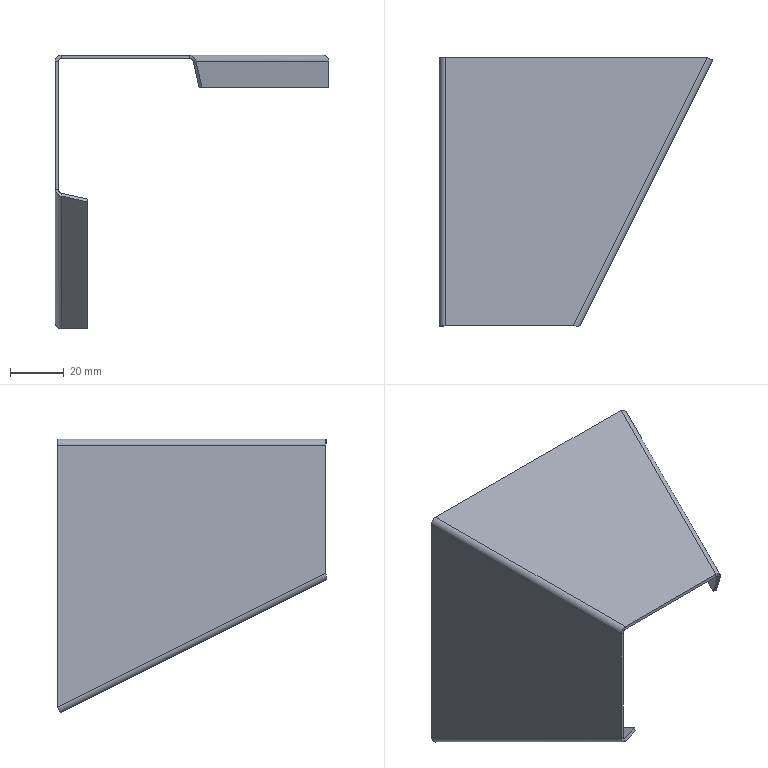Component | SolidWorks | BaseFoot-H100-1 | 1 solid | 30 faces | box 101.97 x 100.16 x 101.97 mm | volume 20988 mm3 | plane 22 | cylinder 6 | spline 2 | commonest cylinder face diameters 2 x3 4.4 x3
STEP:
#1=COLOUR_RGB('',0.7922,0.8196,0.9333);
#2=FILL_AREA_STYLE_COLOUR('',#1);
#3=FILL_AREA_STYLE('',(#2));
#4=SURFACE_STYLE_FILL_AREA(#3);
#5=SURFACE_SIDE_STYLE('',(#4));
#6=SURFACE_STYLE_USAGE(.BOTH.,#5);
#7=PRESENTATION_STYLE_ASSIGNMENT((#6));
#8=CARTESIAN_POINT('',(-19.685,0.,6.102));
#9=VERTEX_POINT('',#8);
#10=CARTESIAN_POINT('',(-19.685,-0.,9.953));
#11=VERTEX_POINT('',#10);
#12=CARTESIAN_POINT('',(-19.685,-0.,6.102));
#13=DIRECTION('',(0.,0.,1.));
#14=VECTOR('',#13,39.37);
#15=LINE('',#12,#14);
#16=EDGE_CURVE('',#9,#11,#15,.T.);
#17=ORIENTED_EDGE('',*,*,#16,.F.);
#18=CARTESIAN_POINT('',(-19.685,-3.937,8.071));
#19=VERTEX_POINT('',#18);
#20=CARTESIAN_POINT('',(-19.685,-3.15,7.677));
#21=DIRECTION('',(-0.,0.8944,-0.4472));
#22=VECTOR('',#21,39.37);
#23=LINE('',#20,#22);
#24=EDGE_CURVE('',#19,#9,#23,.T.);
#25=ORIENTED_EDGE('',*,*,#24,.F.);
#26=CARTESIAN_POINT('',(-19.685,-3.937,9.953));
#27=VERTEX_POINT('',#26);
#28=CARTESIAN_POINT('',(-19.685,-3.937,6.102));
#29=DIRECTION('',(0.,0.,1.));
#30=VECTOR('',#29,39.37);
#31=LINE('',#28,#30);
#32=EDGE_CURVE('',#19,#27,#31,.T.);
#33=ORIENTED_EDGE('',*,*,#32,.T.);
#34=CARTESIAN_POINT('',(-19.685,-3.937,9.953));
#35=DIRECTION('',(0.,1.,0.));
#36=VECTOR('',#35,39.37);
#37=LINE('',#34,#36);
#38=EDGE_CURVE('',#27,#11,#37,.T.);
#39=ORIENTED_EDGE('',*,*,#38,.T.);
#40=EDGE_LOOP('',(#17,#25,#33,#39));
#41=FACE_OUTER_BOUND('',#40,.T.);
#42=CARTESIAN_POINT('',(-19.685,-3.937,6.102));
#43=DIRECTION('',(-1.,0.,0.));
#44=DIRECTION('',(0.,0.,1.));
#45=AXIS2_PLACEMENT_3D('',#42,#43,#44);
#46=PLANE('',#45);
#47=ADVANCED_FACE('',(#41),#46,.T.);
#48=CARTESIAN_POINT('',(-19.638,-3.937,8.071));
#49=VERTEX_POINT('',#48);
#50=CARTESIAN_POINT('',(-19.638,0.,6.102));
#51=VERTEX_POINT('',#50);
#52=CARTESIAN_POINT('',(-19.638,-3.15,7.677));
#53=DIRECTION('',(-0.,0.8944,-0.4472));
#54=VECTOR('',#53,39.37);
#55=LINE('',#52,#54);
#56=EDGE_CURVE('',#49,#51,#55,.T.);
#57=ORIENTED_EDGE('',*,*,#56,.T.);
#58=CARTESIAN_POINT('',(-19.638,-0.,9.953));
#59=VERTEX_POINT('',#58);
#60=CARTESIAN_POINT('',(-19.638,-0.,6.102));
#61=DIRECTION('',(0.,0.,1.));
#62=VECTOR('',#61,39.37);
#63=LINE('',#60,#62);
#64=EDGE_CURVE('',#51,#59,#63,.T.);
#65=ORIENTED_EDGE('',*,*,#64,.T.);
#66=CARTESIAN_POINT('',(-19.638,-3.937,9.953));
#67=VERTEX_POINT('',#66);
#68=CARTESIAN_POINT('',(-19.638,-3.937,9.953));
#69=DIRECTION('',(0.,1.,0.));
#70=VECTOR('',#69,39.37);
#71=LINE('',#68,#70);
#72=EDGE_CURVE('',#67,#59,#71,.T.);
#73=ORIENTED_EDGE('',*,*,#72,.F.);
#74=CARTESIAN_POINT('',(-19.638,-3.937,6.102));
#75=DIRECTION('',(0.,0.,1.));
#76=VECTOR('',#75,39.37);
#77=LINE('',#74,#76);
#78=EDGE_CURVE('',#49,#67,#77,.T.);
#79=ORIENTED_EDGE('',*,*,#78,.F.);
#80=EDGE_LOOP('',(#57,#65,#73,#79));
#81=FACE_OUTER_BOUND('',#80,.T.);
#82=CARTESIAN_POINT('',(-19.638,-3.937,6.102));
#83=DIRECTION('',(-1.,0.,0.));
#84=DIRECTION('',(0.,0.,1.));
#85=AXIS2_PLACEMENT_3D('',#82,#83,#84);
#86=PLANE('',#85);
#87=ADVANCED_FACE('',(#81),#86,.F.);
#88=CARTESIAN_POINT('',(-19.638,-3.937,8.071));
#89=CARTESIAN_POINT('',(-19.685,-3.937,8.071));
#90=B_SPLINE_CURVE_WITH_KNOTS('',1,(#88,#89),.UNSPECIFIED.,.F.,.F.,(2,2),(0.,1.),.UNSPECIFIED.);
#91=EDGE_CURVE('',#49,#19,#90,.T.);
#92=ORIENTED_EDGE('',*,*,#91,.F.);
#93=ORIENTED_EDGE('',*,*,#78,.T.);
#94=CARTESIAN_POINT('',(-19.638,-3.937,9.953));
#95=DIRECTION('',(-1.,0.,0.));
#96=VECTOR('',#95,39.37);
#97=LINE('',#94,#96);
#98=EDGE_CURVE('',#67,#27,#97,.T.);
#99=ORIENTED_EDGE('',*,*,#98,.T.);
#100=ORIENTED_EDGE('',*,*,#32,.F.);
#101=EDGE_LOOP('',(#92,#93,#99,#100));
#102=FACE_OUTER_BOUND('',#101,.T.);
#103=CARTESIAN_POINT('',(-19.598,-3.937,9.953));
#104=DIRECTION('',(0.,1.,0.));
#105=DIRECTION('',(1.,0.,0.));
#106=AXIS2_PLACEMENT_3D('',#103,#104,#105);
#107=PLANE('',#106);
#108=ADVANCED_FACE('',(#102),#107,.F.);
#109=ORIENTED_EDGE('',*,*,#16,.T.);
#110=CARTESIAN_POINT('',(-19.685,-0.,9.953));
#111=DIRECTION('',(1.,0.,-0.));
#112=VECTOR('',#111,39.37);
#113=LINE('',#110,#112);
#114=EDGE_CURVE('',#11,#59,#113,.T.);
#115=ORIENTED_EDGE('',*,*,#114,.T.);
#116=ORIENTED_EDGE('',*,*,#64,.F.);
#117=CARTESIAN_POINT('',(-19.685,-0.,6.102));
#118=DIRECTION('',(1.,0.,0.));
#119=VECTOR('',#118,39.37);
#120=LINE('',#117,#119);
#121=EDGE_CURVE('',#9,#51,#120,.T.);
#122=ORIENTED_EDGE('',*,*,#121,.F.);
#123=EDGE_LOOP('',(#109,#115,#116,#122));
#124=FACE_OUTER_BOUND('',#123,.T.);
#125=CARTESIAN_POINT('',(-19.598,-0.,9.992));
#126=DIRECTION('',(0.,1.,0.));
#127=DIRECTION('',(0.,0.,1.));
#128=AXIS2_PLACEMENT_3D('',#125,#126,#127);
#129=PLANE('',#128);
#130=ADVANCED_FACE('',(#124),#129,.T.);
#131=CARTESIAN_POINT('',(-17.717,-3.937,9.992));
#132=VERTEX_POINT('',#131);
#133=CARTESIAN_POINT('',(-15.748,-0.,9.992));
#134=VERTEX_POINT('',#133);
#135=CARTESIAN_POINT('',(-18.11,-4.724,9.992));
#136=DIRECTION('',(0.4472,0.8944,0.));
#137=VECTOR('',#136,39.37);
#138=LINE('',#135,#137);
#139=EDGE_CURVE('',#132,#134,#138,.T.);
#140=ORIENTED_EDGE('',*,*,#139,.F.);
#141=CARTESIAN_POINT('',(-19.598,-3.937,9.992));
#142=VERTEX_POINT('',#141);
#143=CARTESIAN_POINT('',(-19.685,-3.937,9.992));
#144=DIRECTION('',(1.,0.,0.));
#145=VECTOR('',#144,39.37);
#146=LINE('',#143,#145);
#147=EDGE_CURVE('',#142,#132,#146,.T.);
#148=ORIENTED_EDGE('',*,*,#147,.F.);
#149=CARTESIAN_POINT('',(-19.598,-0.,9.992));
#150=VERTEX_POINT('',#149);
#151=CARTESIAN_POINT('',(-19.598,-3.937,9.992));
#152=DIRECTION('',(0.,1.,0.));
#153=VECTOR('',#152,39.37);
#154=LINE('',#151,#153);
#155=EDGE_CURVE('',#142,#150,#154,.T.);
#156=ORIENTED_EDGE('',*,*,#155,.T.);
#157=CARTESIAN_POINT('',(-19.685,-0.,9.992));
#158=DIRECTION('',(1.,0.,0.));
#159=VECTOR('',#158,39.37);
#160=LINE('',#157,#159);
#161=EDGE_CURVE('',#150,#134,#160,.T.);
#162=ORIENTED_EDGE('',*,*,#161,.T.);
#163=EDGE_LOOP('',(#140,#148,#156,#162));
#164=FACE_OUTER_BOUND('',#163,.T.);
#165=CARTESIAN_POINT('',(-19.685,-3.937,9.992));
#166=DIRECTION('',(0.,0.,1.));
#167=DIRECTION('',(1.,0.,0.));
#168=AXIS2_PLACEMENT_3D('',#165,#166,#167);
#169=PLANE('',#168);
#170=ADVANCED_FACE('',(#164),#169,.F.);
#171=CARTESIAN_POINT('',(-19.598,-0.,10.039));
#172=VERTEX_POINT('',#171);
#173=CARTESIAN_POINT('',(-15.748,-0.,10.039));
#174=VERTEX_POINT('',#173);
#175=CARTESIAN_POINT('',(-19.685,-0.,10.039));
#176=DIRECTION('',(1.,0.,0.));
#177=VECTOR('',#176,39.37);
#178=LINE('',#175,#177);
#179=EDGE_CURVE('',#172,#174,#178,.T.);
#180=ORIENTED_EDGE('',*,*,#179,.T.);
#181=CARTESIAN_POINT('',(-15.748,-0.,9.992));
#182=DIRECTION('',(0.,0.,1.));
#183=VECTOR('',#182,39.37);
#184=LINE('',#181,#183);
#185=EDGE_CURVE('',#134,#174,#184,.T.);
#186=ORIENTED_EDGE('',*,*,#185,.F.);
#187=ORIENTED_EDGE('',*,*,#161,.F.);
#188=CARTESIAN_POINT('',(-19.598,-0.,9.992));
#189=DIRECTION('',(0.,0.,1.));
#190=VECTOR('',#189,39.37);
#191=LINE('',#188,#190);
#192=EDGE_CURVE('',#150,#172,#191,.T.);
#193=ORIENTED_EDGE('',*,*,#192,.T.);
#194=EDGE_LOOP('',(#180,#186,#187,#193));
#195=FACE_OUTER_BOUND('',#194,.T.);
#196=CARTESIAN_POINT('',(-19.598,-0.,9.953));
#197=DIRECTION('',(0.,1.,0.));
#198=DIRECTION('',(1.,0.,0.));
#199=AXIS2_PLACEMENT_3D('',#196,#197,#198);
#200=PLANE('',#199);
#201=ADVANCED_FACE('',(#195),#200,.T.);
#202=CARTESIAN_POINT('',(-19.598,-3.937,10.039));
#203=VERTEX_POINT('',#202);
#204=CARTESIAN_POINT('',(-17.717,-3.937,10.039));
#205=VERTEX_POINT('',#204);
#206=CARTESIAN_POINT('',(-19.685,-3.937,10.039));
#207=DIRECTION('',(1.,0.,0.));
#208=VECTOR('',#207,39.37);
#209=LINE('',#206,#208);
#210=EDGE_CURVE('',#203,#205,#209,.T.);
#211=ORIENTED_EDGE('',*,*,#210,.T.);
#212=CARTESIAN_POINT('',(-18.11,-4.724,10.039));
#213=DIRECTION('',(0.4472,0.8944,0.));
#214=VECTOR('',#213,39.37);
#215=LINE('',#212,#214);
#216=EDGE_CURVE('',#205,#174,#215,.T.);
#217=ORIENTED_EDGE('',*,*,#216,.T.);
#218=ORIENTED_EDGE('',*,*,#179,.F.);
#219=CARTESIAN_POINT('',(-19.598,-3.937,10.039));
#220=DIRECTION('',(0.,1.,0.));
#221=VECTOR('',#220,39.37);
#222=LINE('',#219,#221);
#223=EDGE_CURVE('',#203,#172,#222,.T.);
#224=ORIENTED_EDGE('',*,*,#223,.F.);
#225=EDGE_LOOP('',(#211,#217,#218,#224));
#226=FACE_OUTER_BOUND('',#225,.T.);
#227=CARTESIAN_POINT('',(-19.685,-3.937,10.039));
#228=DIRECTION('',(0.,0.,1.));
#229=DIRECTION('',(1.,0.,0.));
#230=AXIS2_PLACEMENT_3D('',#227,#228,#229);
#231=PLANE('',#230);
#232=ADVANCED_FACE('',(#226),#231,.T.);
#233=ORIENTED_EDGE('',*,*,#147,.T.);
#234=CARTESIAN_POINT('',(-17.717,-3.937,10.039));
#235=CARTESIAN_POINT('',(-17.717,-3.937,9.992));
#236=B_SPLINE_CURVE_WITH_KNOTS('',1,(#234,#235),.UNSPECIFIED.,.F.,.F.,(2,2),(0.,1.),.UNSPECIFIED.);
#237=EDGE_CURVE('',#205,#132,#236,.T.);
#238=ORIENTED_EDGE('',*,*,#237,.F.);
#239=ORIENTED_EDGE('',*,*,#210,.F.);
#240=CARTESIAN_POINT('',(-19.598,-3.937,10.039));
#241=DIRECTION('',(0.,0.,-1.));
#242=VECTOR('',#241,39.37);
#243=LINE('',#240,#242);
#244=EDGE_CURVE('',#203,#142,#243,.T.);
#245=ORIENTED_EDGE('',*,*,#244,.T.);
#246=EDGE_LOOP('',(#233,#238,#239,#245));
#247=FACE_OUTER_BOUND('',#246,.T.);
#248=CARTESIAN_POINT('',(-19.638,-3.937,9.953));
#249=DIRECTION('',(0.,-1.,0.));
#250=DIRECTION('',(0.,0.,-1.));
#251=AXIS2_PLACEMENT_3D('',#248,#249,#250);
#252=PLANE('',#251);
#253=ADVANCED_FACE('',(#247),#252,.T.);
#254=ORIENTED_EDGE('',*,*,#244,.F.);
#255=CARTESIAN_POINT('',(-19.598,-3.937,9.953));
#256=DIRECTION('',(0.,-1.,0.));
#257=DIRECTION('',(0.,0.,1.));
#258=AXIS2_PLACEMENT_3D('',#255,#256,#257);
#259=CIRCLE('',#258,0.08661);
#260=EDGE_CURVE('',#203,#27,#259,.T.);
#261=ORIENTED_EDGE('',*,*,#260,.T.);
#262=ORIENTED_EDGE('',*,*,#98,.F.);
#263=CARTESIAN_POINT('',(-19.598,-3.937,9.953));
#264=DIRECTION('',(0.,-1.,0.));
#265=DIRECTION('',(0.,0.,-1.));
#266=AXIS2_PLACEMENT_3D('',#263,#264,#265);
#267=CIRCLE('',#266,0.03937);
#268=EDGE_CURVE('',#142,#67,#267,.T.);
#269=ORIENTED_EDGE('',*,*,#268,.F.);
#270=EDGE_LOOP('',(#254,#261,#262,#269));
#271=FACE_OUTER_BOUND('',#270,.T.);
#272=CARTESIAN_POINT('',(-19.598,-3.937,9.953));
#273=DIRECTION('',(0.,1.,0.));
#274=DIRECTION('',(0.,0.,1.));
#275=AXIS2_PLACEMENT_3D('',#272,#273,#274);
#276=PLANE('',#275);
#277=ADVANCED_FACE('',(#271),#276,.F.);
#278=ORIENTED_EDGE('',*,*,#114,.F.);
#279=CARTESIAN_POINT('',(-19.598,-0.,9.953));
#280=DIRECTION('',(0.,1.,0.));
#281=DIRECTION('',(0.,0.,1.));
#282=AXIS2_PLACEMENT_3D('',#279,#280,#281);
#283=CIRCLE('',#282,0.08661);
#284=EDGE_CURVE('',#11,#172,#283,.T.);
#285=ORIENTED_EDGE('',*,*,#284,.T.);
#286=ORIENTED_EDGE('',*,*,#192,.F.);
#287=CARTESIAN_POINT('',(-19.598,-0.,9.953));
#288=DIRECTION('',(0.,1.,0.));
#289=DIRECTION('',(0.,0.,1.));
#290=AXIS2_PLACEMENT_3D('',#287,#288,#289);
#291=CIRCLE('',#290,0.03937);
#292=EDGE_CURVE('',#59,#150,#291,.T.);
#293=ORIENTED_EDGE('',*,*,#292,.F.);
#294=EDGE_LOOP('',(#278,#285,#286,#293));
#295=FACE_OUTER_BOUND('',#294,.T.);
#296=CARTESIAN_POINT('',(-19.598,-0.,9.953));
#297=DIRECTION('',(0.,-1.,0.));
#298=DIRECTION('',(0.,0.,-1.));
#299=AXIS2_PLACEMENT_3D('',#296,#297,#298);
#300=PLANE('',#299);
#301=ADVANCED_FACE('',(#295),#300,.F.);
#302=ORIENTED_EDGE('',*,*,#292,.T.);
#303=ORIENTED_EDGE('',*,*,#155,.F.);
#304=ORIENTED_EDGE('',*,*,#268,.T.);
#305=ORIENTED_EDGE('',*,*,#72,.T.);
#306=EDGE_LOOP('',(#302,#303,#304,#305));
#307=FACE_OUTER_BOUND('',#306,.T.);
#308=CARTESIAN_POINT('',(-19.598,-5.907,9.953));
#309=DIRECTION('',(0.,1.,0.));
#310=DIRECTION('',(0.,0.,1.));
#311=AXIS2_PLACEMENT_3D('',#308,#309,#310);
#312=CYLINDRICAL_SURFACE('',#311,0.03937);
#313=ADVANCED_FACE('',(#307),#312,.F.);
#314=ORIENTED_EDGE('',*,*,#284,.F.);
#315=ORIENTED_EDGE('',*,*,#38,.F.);
#316=ORIENTED_EDGE('',*,*,#260,.F.);
#317=ORIENTED_EDGE('',*,*,#223,.T.);
#318=EDGE_LOOP('',(#314,#315,#316,#317));
#319=FACE_OUTER_BOUND('',#318,.T.);
#320=CARTESIAN_POINT('',(-19.598,-5.907,9.953));
#321=DIRECTION('',(0.,1.,0.));
#322=DIRECTION('',(0.,0.,1.));
#323=AXIS2_PLACEMENT_3D('',#320,#321,#322);
#324=CYLINDRICAL_SURFACE('',#323,0.08661);
#325=ADVANCED_FACE('',(#319),#324,.T.);
#326=CARTESIAN_POINT('',(-17.618,-3.933,9.953));
#327=VERTEX_POINT('',#326);
#328=CARTESIAN_POINT('',(-17.66,-3.912,9.953));
#329=VERTEX_POINT('',#328);
#330=CARTESIAN_POINT('',(-17.618,-3.933,9.953));
#331=CARTESIAN_POINT('',(-17.632,-3.926,9.953));
#332=CARTESIAN_POINT('',(-17.646,-3.919,9.953));
#333=CARTESIAN_POINT('',(-17.66,-3.912,9.953));
#334=B_SPLINE_CURVE_WITH_KNOTS('',3,(#330,#331,#332,#333),.UNSPECIFIED.,.F.,.F.,(4,4),(0.,1.),.UNSPECIFIED.);
#335=EDGE_CURVE('',#327,#329,#334,.T.);
#336=ORIENTED_EDGE('',*,*,#335,.F.);
#337=CARTESIAN_POINT('',(-17.618,-3.933,9.953));
#338=CARTESIAN_POINT('',(-17.62,-3.937,9.964));
#339=CARTESIAN_POINT('',(-17.623,-3.94,9.975));
#340=CARTESIAN_POINT('',(-17.635,-3.943,9.996));
#341=CARTESIAN_POINT('',(-17.642,-3.943,10.006));
#342=CARTESIAN_POINT('',(-17.66,-3.943,10.022));
#343=CARTESIAN_POINT('',(-17.67,-3.942,10.028));
#344=CARTESIAN_POINT('',(-17.693,-3.94,10.037));
#345=CARTESIAN_POINT('',(-17.705,-3.939,10.039));
#346=CARTESIAN_POINT('',(-17.717,-3.937,10.039));
#347=B_SPLINE_CURVE_WITH_KNOTS('',3,(#337,#338,#339,#340,#341,#342,#343,#344,#345,#346),.UNSPECIFIED.,.F.,.F.,(4,2,2,2,4),(0.,0.25,0.5,0.75,1.),.UNSPECIFIED.);
#348=EDGE_CURVE('',#327,#205,#347,.T.);
#349=ORIENTED_EDGE('',*,*,#348,.T.);
#350=ORIENTED_EDGE('',*,*,#237,.T.);
#351=CARTESIAN_POINT('',(-17.66,-3.912,9.953));
#352=CARTESIAN_POINT('',(-17.664,-3.919,9.963));
#353=CARTESIAN_POINT('',(-17.671,-3.925,9.973));
#354=CARTESIAN_POINT('',(-17.691,-3.932,9.988));
#355=CARTESIAN_POINT('',(-17.704,-3.935,9.992));
#356=CARTESIAN_POINT('',(-17.717,-3.937,9.992));
#357=B_SPLINE_CURVE_WITH_KNOTS('',3,(#351,#352,#353,#354,#355,#356),.UNSPECIFIED.,.F.,.F.,(4,2,4),(0.,0.5,1.),.UNSPECIFIED.);
#358=EDGE_CURVE('',#329,#132,#357,.T.);
#359=ORIENTED_EDGE('',*,*,#358,.F.);
#360=EDGE_LOOP('',(#336,#349,#350,#359));
#361=FACE_OUTER_BOUND('',#360,.T.);
#362=CARTESIAN_POINT('',(-17.618,-3.933,9.953));
#363=CARTESIAN_POINT('',(-17.62,-3.937,9.964));
#364=CARTESIAN_POINT('',(-17.623,-3.94,9.975));
#365=CARTESIAN_POINT('',(-17.635,-3.943,9.996));
#366=CARTESIAN_POINT('',(-17.642,-3.943,10.006));
#367=CARTESIAN_POINT('',(-17.66,-3.943,10.022));
#368=CARTESIAN_POINT('',(-17.67,-3.942,10.028));
#369=CARTESIAN_POINT('',(-17.693,-3.94,10.037));
#370=CARTESIAN_POINT('',(-17.705,-3.939,10.039));
#371=CARTESIAN_POINT('',(-17.717,-3.937,10.039));
#372=CARTESIAN_POINT('',(-17.66,-3.912,9.953));
#373=CARTESIAN_POINT('',(-17.662,-3.916,9.958));
#374=CARTESIAN_POINT('',(-17.665,-3.919,9.963));
#375=CARTESIAN_POINT('',(-17.672,-3.924,9.973));
#376=CARTESIAN_POINT('',(-17.676,-3.926,9.977));
#377=CARTESIAN_POINT('',(-17.686,-3.93,9.984));
#378=CARTESIAN_POINT('',(-17.692,-3.932,9.987));
#379=CARTESIAN_POINT('',(-17.704,-3.935,9.991));
#380=CARTESIAN_POINT('',(-17.71,-3.936,9.992));
#381=CARTESIAN_POINT('',(-17.717,-3.937,9.992));
#382=B_SPLINE_SURFACE_WITH_KNOTS('',1,3,((#362,#363,#364,#365,#366,#367,#368,#369,#370,#371),(#372,#373,#374,#375,#376,#377,#378,#379,#380,#381)),.UNSPECIFIED.,.F.,.F.,.F.,(2,2),(4,2,2,2,4),(0.,1.),(0.,0.25,0.5,0.75,1.),.UNSPECIFIED.);
#383=ADVANCED_FACE('',(#361),#382,.F.);
#384=CARTESIAN_POINT('',(-15.671,-0.03874,9.953));
#385=VERTEX_POINT('',#384);
#386=CARTESIAN_POINT('',(-15.748,0.,9.953));
#387=DIRECTION('',(0.4472,0.8944,0.));
#388=DIRECTION('',(0.8944,-0.4472,0.));
#389=AXIS2_PLACEMENT_3D('',#386,#387,#388);
#390=CIRCLE('',#389,0.08661);
#391=EDGE_CURVE('',#174,#385,#390,.T.);
#392=ORIENTED_EDGE('',*,*,#391,.T.);
#393=CARTESIAN_POINT('',(-15.713,-0.01761,9.953));
#394=VERTEX_POINT('',#393);
#395=CARTESIAN_POINT('',(-15.671,-0.03874,9.953));
#396=DIRECTION('',(0.8944,-0.4472,0.));
#397=VECTOR('',#396,39.37);
#398=LINE('',#395,#397);
#399=EDGE_CURVE('',#394,#385,#398,.T.);
#400=ORIENTED_EDGE('',*,*,#399,.F.);
#401=CARTESIAN_POINT('',(-15.748,0.,9.953));
#402=DIRECTION('',(0.4472,0.8944,0.));
#403=DIRECTION('',(-0.8944,0.4472,0.));
#404=AXIS2_PLACEMENT_3D('',#401,#402,#403);
#405=CIRCLE('',#404,0.03937);
#406=EDGE_CURVE('',#134,#394,#405,.T.);
#407=ORIENTED_EDGE('',*,*,#406,.F.);
#408=ORIENTED_EDGE('',*,*,#185,.T.);
#409=EDGE_LOOP('',(#392,#400,#407,#408));
#410=FACE_OUTER_BOUND('',#409,.T.);
#411=CARTESIAN_POINT('',(-15.748,0.,9.953));
#412=DIRECTION('',(-0.4472,-0.8944,-0.));
#413=DIRECTION('',(0.8944,-0.4472,0.));
#414=AXIS2_PLACEMENT_3D('',#411,#412,#413);
#415=PLANE('',#414);
#416=ADVANCED_FACE('',(#410),#415,.F.);
#417=ORIENTED_EDGE('',*,*,#139,.T.);
#418=ORIENTED_EDGE('',*,*,#406,.T.);
#419=CARTESIAN_POINT('',(-15.713,-0.01761,9.953));
#420=DIRECTION('',(-0.4472,-0.8944,0.));
#421=VECTOR('',#420,39.37);
#422=LINE('',#419,#421);
#423=EDGE_CURVE('',#394,#329,#422,.T.);
#424=ORIENTED_EDGE('',*,*,#423,.T.);
#425=ORIENTED_EDGE('',*,*,#358,.T.);
#426=EDGE_LOOP('',(#417,#418,#424,#425));
#427=FACE_OUTER_BOUND('',#426,.T.);
#428=CARTESIAN_POINT('',(-14.746,2.003,9.953));
#429=DIRECTION('',(-0.4472,-0.8944,0.));
#430=DIRECTION('',(0.8944,-0.4472,0.));
#431=AXIS2_PLACEMENT_3D('',#428,#429,#430);
#432=CYLINDRICAL_SURFACE('',#431,0.03937);
#433=ADVANCED_FACE('',(#427),#432,.F.);
#434=ORIENTED_EDGE('',*,*,#216,.F.);
#435=ORIENTED_EDGE('',*,*,#348,.F.);
#436=CARTESIAN_POINT('',(-16.458,-1.614,9.953));
#437=DIRECTION('',(-0.4472,-0.8944,0.));
#438=VECTOR('',#437,39.37);
#439=LINE('',#436,#438);
#440=EDGE_CURVE('',#385,#327,#439,.T.);
#441=ORIENTED_EDGE('',*,*,#440,.F.);
#442=ORIENTED_EDGE('',*,*,#391,.F.);
#443=EDGE_LOOP('',(#434,#435,#441,#442));
#444=FACE_OUTER_BOUND('',#443,.T.);
#445=CARTESIAN_POINT('',(-14.746,2.003,9.953));
#446=DIRECTION('',(-0.4472,-0.8944,0.));
#447=DIRECTION('',(0.8944,-0.4472,0.));
#448=AXIS2_PLACEMENT_3D('',#445,#446,#447);
#449=CYLINDRICAL_SURFACE('',#448,0.08661);
#450=ADVANCED_FACE('',(#444),#449,.T.);
#451=CARTESIAN_POINT('',(-15.671,-0.03874,9.567));
#452=VERTEX_POINT('',#451);
#453=CARTESIAN_POINT('',(-17.532,-3.761,9.567));
#454=VERTEX_POINT('',#453);
#455=CARTESIAN_POINT('',(-17.639,-3.976,9.567));
#456=DIRECTION('',(-0.4472,-0.8944,0.));
#457=VECTOR('',#456,39.37);
#458=LINE('',#455,#457);
#459=EDGE_CURVE('',#452,#454,#458,.T.);
#460=ORIENTED_EDGE('',*,*,#459,.T.);
#461=CARTESIAN_POINT('',(-17.574,-3.74,9.567));
#462=VERTEX_POINT('',#461);
#463=CARTESIAN_POINT('',(-17.532,-3.761,9.567));
#464=DIRECTION('',(-0.8944,0.4472,-0.));
#465=VECTOR('',#464,39.37);
#466=LINE('',#463,#465);
#467=EDGE_CURVE('',#454,#462,#466,.T.);
#468=ORIENTED_EDGE('',*,*,#467,.T.);
#469=CARTESIAN_POINT('',(-15.713,-0.01761,9.567));
#470=VERTEX_POINT('',#469);
#471=CARTESIAN_POINT('',(-16.5,-1.592,9.567));
#472=DIRECTION('',(-0.4472,-0.8944,0.));
#473=VECTOR('',#472,39.37);
#474=LINE('',#471,#473);
#475=EDGE_CURVE('',#470,#462,#474,.T.);
#476=ORIENTED_EDGE('',*,*,#475,.F.);
#477=CARTESIAN_POINT('',(-15.671,-0.03874,9.567));
#478=DIRECTION('',(-0.8944,0.4472,-0.));
#479=VECTOR('',#478,39.37);
#480=LINE('',#477,#479);
#481=EDGE_CURVE('',#452,#470,#480,.T.);
#482=ORIENTED_EDGE('',*,*,#481,.F.);
#483=EDGE_LOOP('',(#460,#468,#476,#482));
#484=FACE_OUTER_BOUND('',#483,.T.);
#485=CARTESIAN_POINT('',(-17.639,-3.976,9.567));
#486=DIRECTION('',(0.,-0.,-1.));
#487=DIRECTION('',(-1.,-0.,-0.));
#488=AXIS2_PLACEMENT_3D('',#485,#486,#487);
#489=PLANE('',#488);
#490=ADVANCED_FACE('',(#484),#489,.T.);
#491=CARTESIAN_POINT('',(-17.444,-3.479,8.985));
#492=DIRECTION('',(-0.2,-0.4,0.8944));
#493=VECTOR('',#492,39.37);
#494=LINE('',#491,#493);
#495=EDGE_CURVE('',#462,#329,#494,.T.);
#496=ORIENTED_EDGE('',*,*,#495,.T.);
#497=ORIENTED_EDGE('',*,*,#423,.F.);
#498=CARTESIAN_POINT('',(-15.713,-0.01761,10.039));
#499=DIRECTION('',(0.,0.,-1.));
#500=VECTOR('',#499,39.37);
#501=LINE('',#498,#500);
#502=EDGE_CURVE('',#394,#470,#501,.T.);
#503=ORIENTED_EDGE('',*,*,#502,.T.);
#504=ORIENTED_EDGE('',*,*,#475,.T.);
#505=EDGE_LOOP('',(#496,#497,#503,#504));
#506=FACE_OUTER_BOUND('',#505,.T.);
#507=CARTESIAN_POINT('',(-16.5,-1.592,10.039));
#508=DIRECTION('',(0.8944,-0.4472,0.));
#509=DIRECTION('',(0.4472,0.8944,-0.));
#510=AXIS2_PLACEMENT_3D('',#507,#508,#509);
#511=PLANE('',#510);
#512=ADVANCED_FACE('',(#506),#511,.F.);
#513=ORIENTED_EDGE('',*,*,#502,.F.);
#514=ORIENTED_EDGE('',*,*,#399,.T.);
#515=CARTESIAN_POINT('',(-15.671,-0.03874,9.567));
#516=DIRECTION('',(0.,0.,-1.));
#517=VECTOR('',#516,39.37);
#518=LINE('',#515,#517);
#519=EDGE_CURVE('',#385,#452,#518,.T.);
#520=ORIENTED_EDGE('',*,*,#519,.T.);
#521=ORIENTED_EDGE('',*,*,#481,.T.);
#522=EDGE_LOOP('',(#513,#514,#520,#521));
#523=FACE_OUTER_BOUND('',#522,.T.);
#524=CARTESIAN_POINT('',(-15.671,-0.03874,9.567));
#525=DIRECTION('',(0.4472,0.8944,0.));
#526=DIRECTION('',(-0.8944,0.4472,-0.));
#527=AXIS2_PLACEMENT_3D('',#524,#525,#526);
#528=PLANE('',#527);
#529=ADVANCED_FACE('',(#523),#528,.T.);
#530=ORIENTED_EDGE('',*,*,#440,.T.);
#531=CARTESIAN_POINT('',(-17.401,-3.5,8.985));
#532=DIRECTION('',(-0.2,-0.4,0.8944));
#533=VECTOR('',#532,39.37);
#534=LINE('',#531,#533);
#535=EDGE_CURVE('',#454,#327,#534,.T.);
#536=ORIENTED_EDGE('',*,*,#535,.F.);
#537=ORIENTED_EDGE('',*,*,#459,.F.);
#538=ORIENTED_EDGE('',*,*,#519,.F.);
#539=EDGE_LOOP('',(#530,#536,#537,#538));
#540=FACE_OUTER_BOUND('',#539,.T.);
#541=CARTESIAN_POINT('',(-16.458,-1.614,10.039));
#542=DIRECTION('',(0.8944,-0.4472,0.));
#543=DIRECTION('',(0.4472,0.8944,-0.));
#544=AXIS2_PLACEMENT_3D('',#541,#542,#543);
#545=PLANE('',#544);
#546=ADVANCED_FACE('',(#540),#545,.T.);
#547=ORIENTED_EDGE('',*,*,#535,.T.);
#548=ORIENTED_EDGE('',*,*,#335,.T.);
#549=ORIENTED_EDGE('',*,*,#495,.F.);
#550=ORIENTED_EDGE('',*,*,#467,.F.);
#551=EDGE_LOOP('',(#547,#548,#549,#550));
#552=FACE_OUTER_BOUND('',#551,.T.);
#553=CARTESIAN_POINT('',(-17.401,-3.5,8.985));
#554=DIRECTION('',(0.4,0.8,0.4472));
#555=DIRECTION('',(-0.2,-0.4,0.8944));
#556=AXIS2_PLACEMENT_3D('',#553,#554,#555);
#557=PLANE('',#556);
#558=ADVANCED_FACE('',(#552),#557,.F.);
#559=ORIENTED_EDGE('',*,*,#91,.T.);
#560=CARTESIAN_POINT('',(-19.598,-3.933,7.972));
#561=VERTEX_POINT('',#560);
#562=CARTESIAN_POINT('',(-19.685,-3.937,8.071));
#563=CARTESIAN_POINT('',(-19.685,-3.939,8.059));
#564=CARTESIAN_POINT('',(-19.683,-3.94,8.047));
#565=CARTESIAN_POINT('',(-19.674,-3.942,8.025));
#566=CARTESIAN_POINT('',(-19.668,-3.943,8.014));
#567=CARTESIAN_POINT('',(-19.652,-3.943,7.997));
#568=CARTESIAN_POINT('',(-19.642,-3.943,7.989));
#569=CARTESIAN_POINT('',(-19.621,-3.94,7.978));
#570=CARTESIAN_POINT('',(-19.61,-3.937,7.974));
#571=CARTESIAN_POINT('',(-19.598,-3.933,7.972));
#572=B_SPLINE_CURVE_WITH_KNOTS('',3,(#562,#563,#564,#565,#566,#567,#568,#569,#570,#571),.UNSPECIFIED.,.F.,.F.,(4,2,2,2,4),(0.,0.25,0.5,0.75,1.),.UNSPECIFIED.);
#573=EDGE_CURVE('',#19,#561,#572,.T.);
#574=ORIENTED_EDGE('',*,*,#573,.T.);
#575=CARTESIAN_POINT('',(-19.598,-3.912,8.015));
#576=VERTEX_POINT('',#575);
#577=CARTESIAN_POINT('',(-19.598,-3.912,8.015));
#578=CARTESIAN_POINT('',(-19.598,-3.919,8.));
#579=CARTESIAN_POINT('',(-19.598,-3.926,7.986));
#580=CARTESIAN_POINT('',(-19.598,-3.933,7.972));
#581=B_SPLINE_CURVE_WITH_KNOTS('',3,(#577,#578,#579,#580),.UNSPECIFIED.,.F.,.F.,(4,4),(0.,1.),.UNSPECIFIED.);
#582=EDGE_CURVE('',#576,#561,#581,.T.);
#583=ORIENTED_EDGE('',*,*,#582,.F.);
#584=CARTESIAN_POINT('',(-19.638,-3.937,8.071));
#585=CARTESIAN_POINT('',(-19.638,-3.935,8.058));
#586=CARTESIAN_POINT('',(-19.634,-3.932,8.045));
#587=CARTESIAN_POINT('',(-19.619,-3.925,8.025));
#588=CARTESIAN_POINT('',(-19.609,-3.919,8.018));
#589=CARTESIAN_POINT('',(-19.598,-3.912,8.015));
#590=B_SPLINE_CURVE_WITH_KNOTS('',3,(#584,#585,#586,#587,#588,#589),.UNSPECIFIED.,.F.,.F.,(4,2,4),(0.,0.5,1.),.UNSPECIFIED.);
#591=EDGE_CURVE('',#49,#576,#590,.T.);
#592=ORIENTED_EDGE('',*,*,#591,.F.);
#593=EDGE_LOOP('',(#559,#574,#583,#592));
#594=FACE_OUTER_BOUND('',#593,.T.);
#595=CARTESIAN_POINT('',(-19.685,-3.937,8.071));
#596=CARTESIAN_POINT('',(-19.685,-3.939,8.059));
#597=CARTESIAN_POINT('',(-19.683,-3.94,8.047));
#598=CARTESIAN_POINT('',(-19.674,-3.942,8.025));
#599=CARTESIAN_POINT('',(-19.668,-3.943,8.014));
#600=CARTESIAN_POINT('',(-19.652,-3.943,7.997));
#601=CARTESIAN_POINT('',(-19.642,-3.943,7.989));
#602=CARTESIAN_POINT('',(-19.621,-3.94,7.978));
#603=CARTESIAN_POINT('',(-19.61,-3.937,7.974));
#604=CARTESIAN_POINT('',(-19.598,-3.933,7.972));
#605=CARTESIAN_POINT('',(-19.638,-3.937,8.071));
#606=CARTESIAN_POINT('',(-19.638,-3.936,8.064));
#607=CARTESIAN_POINT('',(-19.637,-3.935,8.058));
#608=CARTESIAN_POINT('',(-19.633,-3.932,8.046));
#609=CARTESIAN_POINT('',(-19.63,-3.93,8.04));
#610=CARTESIAN_POINT('',(-19.623,-3.926,8.03));
#611=CARTESIAN_POINT('',(-19.618,-3.924,8.026));
#612=CARTESIAN_POINT('',(-19.609,-3.919,8.019));
#613=CARTESIAN_POINT('',(-19.604,-3.916,8.016));
#614=CARTESIAN_POINT('',(-19.598,-3.912,8.015));
#615=B_SPLINE_SURFACE_WITH_KNOTS('',1,3,((#595,#596,#597,#598,#599,#600,#601,#602,#603,#604),(#605,#606,#607,#608,#609,#610,#611,#612,#613,#614)),.UNSPECIFIED.,.F.,.F.,.F.,(2,2),(4,2,2,2,4),(0.,1.),(0.,0.25,0.5,0.75,1.),.UNSPECIFIED.);
#616=ADVANCED_FACE('',(#594),#615,.F.);
#617=CARTESIAN_POINT('',(-19.598,-0.03874,6.025));
#618=VERTEX_POINT('',#617);
#619=CARTESIAN_POINT('',(-19.598,0.,6.102));
#620=DIRECTION('',(-0.,0.8944,-0.4472));
#621=DIRECTION('',(0.,0.4472,0.8944));
#622=AXIS2_PLACEMENT_3D('',#619,#620,#621);
#623=CIRCLE('',#622,0.08661);
#624=EDGE_CURVE('',#618,#9,#623,.T.);
#625=ORIENTED_EDGE('',*,*,#624,.T.);
#626=ORIENTED_EDGE('',*,*,#121,.T.);
#627=CARTESIAN_POINT('',(-19.598,-0.01761,6.067));
#628=VERTEX_POINT('',#627);
#629=CARTESIAN_POINT('',(-19.598,0.,6.102));
#630=DIRECTION('',(0.,0.8944,-0.4472));
#631=DIRECTION('',(0.,0.4472,0.8944));
#632=AXIS2_PLACEMENT_3D('',#629,#630,#631);
#633=CIRCLE('',#632,0.03937);
#634=EDGE_CURVE('',#628,#51,#633,.T.);
#635=ORIENTED_EDGE('',*,*,#634,.F.);
#636=CARTESIAN_POINT('',(-19.598,-0.01761,6.067));
#637=DIRECTION('',(-0.,-0.4472,-0.8944));
#638=VECTOR('',#637,39.37);
#639=LINE('',#636,#638);
#640=EDGE_CURVE('',#628,#618,#639,.T.);
#641=ORIENTED_EDGE('',*,*,#640,.T.);
#642=EDGE_LOOP('',(#625,#626,#635,#641));
#643=FACE_OUTER_BOUND('',#642,.T.);
#644=CARTESIAN_POINT('',(-19.598,0.,6.102));
#645=DIRECTION('',(-0.,-0.8944,0.4472));
#646=DIRECTION('',(0.,-0.4472,-0.8944));
#647=AXIS2_PLACEMENT_3D('',#644,#645,#646);
#648=PLANE('',#647);
#649=ADVANCED_FACE('',(#643),#648,.F.);
#650=CARTESIAN_POINT('',(-19.598,-3.955,8.036));
#651=DIRECTION('',(0.,0.8944,-0.4472));
#652=VECTOR('',#651,39.37);
#653=LINE('',#650,#652);
#654=EDGE_CURVE('',#576,#628,#653,.T.);
#655=ORIENTED_EDGE('',*,*,#654,.T.);
#656=ORIENTED_EDGE('',*,*,#634,.T.);
#657=ORIENTED_EDGE('',*,*,#56,.F.);
#658=ORIENTED_EDGE('',*,*,#591,.T.);
#659=EDGE_LOOP('',(#655,#656,#657,#658));
#660=FACE_OUTER_BOUND('',#659,.T.);
#661=CARTESIAN_POINT('',(-19.598,-5.94,9.072));
#662=DIRECTION('',(-0.,0.8944,-0.4472));
#663=DIRECTION('',(0.,0.4472,0.8944));
#664=AXIS2_PLACEMENT_3D('',#661,#662,#663);
#665=CYLINDRICAL_SURFACE('',#664,0.03937);
#666=ADVANCED_FACE('',(#660),#665,.F.);
#667=CARTESIAN_POINT('',(-19.598,-3.976,7.993));
#668=DIRECTION('',(-0.,-0.8944,0.4472));
#669=VECTOR('',#668,39.37);
#670=LINE('',#667,#669);
#671=EDGE_CURVE('',#618,#561,#670,.T.);
#672=ORIENTED_EDGE('',*,*,#671,.T.);
#673=ORIENTED_EDGE('',*,*,#573,.F.);
#674=ORIENTED_EDGE('',*,*,#24,.T.);
#675=ORIENTED_EDGE('',*,*,#624,.F.);
#676=EDGE_LOOP('',(#672,#673,#674,#675));
#677=FACE_OUTER_BOUND('',#676,.T.);
#678=CARTESIAN_POINT('',(-19.598,-5.94,9.072));
#679=DIRECTION('',(-0.,0.8944,-0.4472));
#680=DIRECTION('',(0.,0.4472,0.8944));
#681=AXIS2_PLACEMENT_3D('',#678,#679,#680);
#682=CYLINDRICAL_SURFACE('',#681,0.08661);
#683=ADVANCED_FACE('',(#677),#682,.T.);
#684=CARTESIAN_POINT('',(-19.213,-3.74,7.928));
#685=VERTEX_POINT('',#684);
#686=CARTESIAN_POINT('',(-19.213,-0.01761,6.067));
#687=VERTEX_POINT('',#686);
#688=CARTESIAN_POINT('',(-19.213,-1.592,6.855));
#689=DIRECTION('',(-0.,0.8944,-0.4472));
#690=VECTOR('',#689,39.37);
#691=LINE('',#688,#690);
#692=EDGE_CURVE('',#685,#687,#691,.T.);
#693=ORIENTED_EDGE('',*,*,#692,.F.);
#694=CARTESIAN_POINT('',(-19.213,-3.761,7.886));
#695=VERTEX_POINT('',#694);
#696=CARTESIAN_POINT('',(-19.213,-3.74,7.928));
#697=DIRECTION('',(-0.,-0.4472,-0.8944));
#698=VECTOR('',#697,39.37);
#699=LINE('',#696,#698);
#700=EDGE_CURVE('',#685,#695,#699,.T.);
#701=ORIENTED_EDGE('',*,*,#700,.T.);
#702=CARTESIAN_POINT('',(-19.213,-0.03874,6.025));
#703=VERTEX_POINT('',#702);
#704=CARTESIAN_POINT('',(-19.213,-3.976,7.993));
#705=DIRECTION('',(-0.,0.8944,-0.4472));
#706=VECTOR('',#705,39.37);
#707=LINE('',#704,#706);
#708=EDGE_CURVE('',#695,#703,#707,.T.);
#709=ORIENTED_EDGE('',*,*,#708,.T.);
#710=CARTESIAN_POINT('',(-19.213,-0.03874,6.025));
#711=DIRECTION('',(0.,0.4472,0.8944));
#712=VECTOR('',#711,39.37);
#713=LINE('',#710,#712);
#714=EDGE_CURVE('',#703,#687,#713,.T.);
#715=ORIENTED_EDGE('',*,*,#714,.T.);
#716=EDGE_LOOP('',(#693,#701,#709,#715));
#717=FACE_OUTER_BOUND('',#716,.T.);
#718=CARTESIAN_POINT('',(-19.213,-3.976,7.993));
#719=DIRECTION('',(1.,-0.,-0.));
#720=DIRECTION('',(-0.,0.,-1.));
#721=AXIS2_PLACEMENT_3D('',#718,#719,#720);
#722=PLANE('',#721);
#723=ADVANCED_FACE('',(#717),#722,.T.);
#724=ORIENTED_EDGE('',*,*,#654,.F.);
#725=CARTESIAN_POINT('',(-18.63,-3.479,7.798));
#726=DIRECTION('',(-0.8944,-0.4,0.2));
#727=VECTOR('',#726,39.37);
#728=LINE('',#725,#727);
#729=EDGE_CURVE('',#685,#576,#728,.T.);
#730=ORIENTED_EDGE('',*,*,#729,.F.);
#731=ORIENTED_EDGE('',*,*,#692,.T.);
#732=CARTESIAN_POINT('',(-19.685,-0.01761,6.067));
#733=DIRECTION('',(-1.,0.,0.));
#734=VECTOR('',#733,39.37);
#735=LINE('',#732,#734);
#736=EDGE_CURVE('',#687,#628,#735,.T.);
#737=ORIENTED_EDGE('',*,*,#736,.T.);
#738=EDGE_LOOP('',(#724,#730,#731,#737));
#739=FACE_OUTER_BOUND('',#738,.T.);
#740=CARTESIAN_POINT('',(-19.685,-1.592,6.855));
#741=DIRECTION('',(0.,0.4472,0.8944));
#742=DIRECTION('',(-0.,-0.8944,0.4472));
#743=AXIS2_PLACEMENT_3D('',#740,#741,#742);
#744=PLANE('',#743);
#745=ADVANCED_FACE('',(#739),#744,.T.);
#746=ORIENTED_EDGE('',*,*,#729,.T.);
#747=ORIENTED_EDGE('',*,*,#582,.T.);
#748=CARTESIAN_POINT('',(-18.63,-3.5,7.756));
#749=DIRECTION('',(-0.8944,-0.4,0.2));
#750=VECTOR('',#749,39.37);
#751=LINE('',#748,#750);
#752=EDGE_CURVE('',#695,#561,#751,.T.);
#753=ORIENTED_EDGE('',*,*,#752,.F.);
#754=ORIENTED_EDGE('',*,*,#700,.F.);
#755=EDGE_LOOP('',(#746,#747,#753,#754));
#756=FACE_OUTER_BOUND('',#755,.T.);
#757=CARTESIAN_POINT('',(-18.63,-3.479,7.798));
#758=DIRECTION('',(-0.4472,0.8,-0.4));
#759=DIRECTION('',(-0.8944,-0.4,0.2));
#760=AXIS2_PLACEMENT_3D('',#757,#758,#759);
#761=PLANE('',#760);
#762=ADVANCED_FACE('',(#756),#761,.F.);
#763=ORIENTED_EDGE('',*,*,#752,.T.);
#764=ORIENTED_EDGE('',*,*,#671,.F.);
#765=CARTESIAN_POINT('',(-19.213,-0.03874,6.025));
#766=DIRECTION('',(-1.,0.,0.));
#767=VECTOR('',#766,39.37);
#768=LINE('',#765,#767);
#769=EDGE_CURVE('',#703,#618,#768,.T.);
#770=ORIENTED_EDGE('',*,*,#769,.F.);
#771=ORIENTED_EDGE('',*,*,#708,.F.);
#772=EDGE_LOOP('',(#763,#764,#770,#771));
#773=FACE_OUTER_BOUND('',#772,.T.);
#774=CARTESIAN_POINT('',(-19.685,-1.614,6.812));
#775=DIRECTION('',(0.,0.4472,0.8944));
#776=DIRECTION('',(-0.,-0.8944,0.4472));
#777=AXIS2_PLACEMENT_3D('',#774,#775,#776);
#778=PLANE('',#777);
#779=ADVANCED_FACE('',(#773),#778,.F.);
#780=ORIENTED_EDGE('',*,*,#769,.T.);
#781=ORIENTED_EDGE('',*,*,#640,.F.);
#782=ORIENTED_EDGE('',*,*,#736,.F.);
#783=ORIENTED_EDGE('',*,*,#714,.F.);
#784=EDGE_LOOP('',(#780,#781,#782,#783));
#785=FACE_OUTER_BOUND('',#784,.T.);
#786=CARTESIAN_POINT('',(-19.213,-0.03874,6.025));
#787=DIRECTION('',(0.,0.8944,-0.4472));
#788=DIRECTION('',(0.,0.4472,0.8944));
#789=AXIS2_PLACEMENT_3D('',#786,#787,#788);
#790=PLANE('',#789);
#791=ADVANCED_FACE('',(#785),#790,.T.);
#792=CLOSED_SHELL('',(#47,#87,#108,#130,#170,#201,#232,#253,#277,#301,#313,#325,#383,#416,#433,#450,#490,#512,#529,#546,#558,#616,#649,#666,#683,#723,#745,#762,#779,#791));
#793=MANIFOLD_SOLID_BREP('',#792);
#794=STYLED_ITEM('',(#7),#793);
#795=(LENGTH_UNIT()NAMED_UNIT(*)SI_UNIT($,.METRE.));
#796=LENGTH_MEASURE_WITH_UNIT(LENGTH_MEASURE(0.0254),#795);
#797=DIMENSIONAL_EXPONENTS(1.,0.,0.,0.,0.,0.,0.);
#798=(CONVERSION_BASED_UNIT('',#796)LENGTH_UNIT()NAMED_UNIT(#797));
#799=UNCERTAINTY_MEASURE_WITH_UNIT(LENGTH_MEASURE(0.00001),#798,'','');
#800=(NAMED_UNIT(*)PLANE_ANGLE_UNIT()SI_UNIT($,.RADIAN.));
#801=(NAMED_UNIT(*)SI_UNIT($,.STERADIAN.)SOLID_ANGLE_UNIT());
#802=(GEOMETRIC_REPRESENTATION_CONTEXT(3)GLOBAL_UNCERTAINTY_ASSIGNED_CONTEXT((#799))GLOBAL_UNIT_ASSIGNED_CONTEXT((#798,#800,#801))REPRESENTATION_CONTEXT('',''));
#803=MECHANICAL_DESIGN_GEOMETRIC_PRESENTATION_REPRESENTATION('',(#794),#802);
#804=CARTESIAN_POINT('',(0.,0.,0.));
#805=DIRECTION('',(0.,0.,1.));
#806=DIRECTION('',(1.,0.,0.));
#807=AXIS2_PLACEMENT_3D('',#804,#805,#806);
#808=(LENGTH_UNIT()NAMED_UNIT(*)SI_UNIT($,.METRE.));
#809=LENGTH_MEASURE_WITH_UNIT(LENGTH_MEASURE(0.0254),#808);
#810=DIMENSIONAL_EXPONENTS(1.,0.,0.,0.,0.,0.,0.);
#811=(CONVERSION_BASED_UNIT('',#809)LENGTH_UNIT()NAMED_UNIT(#810));
#812=UNCERTAINTY_MEASURE_WITH_UNIT(LENGTH_MEASURE(0.00001),#811,'','');
#813=(NAMED_UNIT(*)PLANE_ANGLE_UNIT()SI_UNIT($,.RADIAN.));
#814=(NAMED_UNIT(*)SI_UNIT($,.STERADIAN.)SOLID_ANGLE_UNIT());
#815=(GEOMETRIC_REPRESENTATION_CONTEXT(3)GLOBAL_UNCERTAINTY_ASSIGNED_CONTEXT((#812))GLOBAL_UNIT_ASSIGNED_CONTEXT((#811,#813,#814))REPRESENTATION_CONTEXT('',''));
#816=ADVANCED_BREP_SHAPE_REPRESENTATION('',(#793,#807),#815);
#817=PRESENTATION_LAYER_ASSIGNMENT('','',(#794));